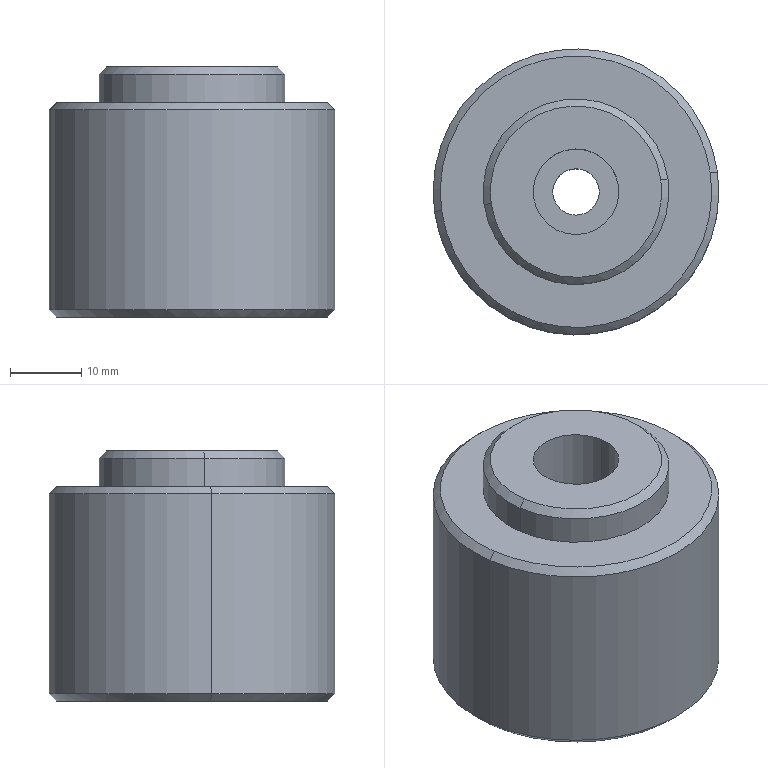Component | SolidWorks | TAR-02-030CoarseKnurledHandwheel-1 | 1 solid | 21 faces | box 40 x 40 x 35 mm | volume 37397 mm3 | cylinder 10 | cone 6 | plane 5 | commonest cylinder face diameters 11 x2 12 x2 26 x2 40 x2 6.5 x2
build123d program:
from build123d import *

# Parameters (mm, degrees)
SKETCH1_R           = 20
BOSS_EXTRUDE1_DEPTH = 30
SKETCH2_R           = 13
BOSS_EXTRUDE2_DEPTH = 5
SKETCH3_R           = 6
CUT_EXTRUDE1_DEPTH  = 15
SKETCH4_R           = 3.25
CUT_EXTRUDE2_DEPTH  = 99
SKETCH5_R           = 5.5
CUT_EXTRUDE3_DEPTH  = 7
CHAMFER1_SIZE       = 1


with BuildPart() as part:
    # Sketch1 → Boss-Extrude1 (new body)
    with BuildSketch(Plane.XY):
        Circle(SKETCH1_R)
    extrude(amount=BOSS_EXTRUDE1_DEPTH)

    # Sketch2 → Boss-Extrude2 (add)
    with BuildSketch(Plane.XY.offset(30)):
        Circle(SKETCH2_R)
    extrude(amount=BOSS_EXTRUDE2_DEPTH)

    # Sketch3 → Cut-Extrude1 (cut)
    with BuildSketch(Plane.XY.offset(35)):
        Circle(SKETCH3_R)
    extrude(amount=-CUT_EXTRUDE1_DEPTH, mode=Mode.SUBTRACT)

    # Sketch4 → Cut-Extrude2 (cut)
    with BuildSketch(Plane.XY.offset(20)):
        Circle(SKETCH4_R)
    extrude(amount=-CUT_EXTRUDE2_DEPTH, mode=Mode.SUBTRACT)

    # Sketch5 → Cut-Extrude3 (cut)
    with BuildSketch(Plane(origin=(0, 0, 0), x_dir=(-1, 0, 0), z_dir=(0, 0, -1))):
        Circle(SKETCH5_R)
    extrude(amount=-CUT_EXTRUDE3_DEPTH, mode=Mode.SUBTRACT)

    # Chamfer1
    chamfer1_edges = [part.edges().sort_by_distance(p)[0] for p in [
        (-20, 0, 0),
        (-20, 0, 30),
        (-13, 0, 35),
    ]]
    chamfer(chamfer1_edges, length=CHAMFER1_SIZE)


solid = part.part

# Placed as in the assembly
solid = solid.moved(Location((14.609, 9.288, -212.6), (0, 0, 0)))
STEP:
#1=COLOUR_RGB('',0.7922,0.8196,0.9333);
#2=FILL_AREA_STYLE_COLOUR('',#1);
#3=FILL_AREA_STYLE('',(#2));
#4=SURFACE_STYLE_FILL_AREA(#3);
#5=SURFACE_SIDE_STYLE('',(#4));
#6=SURFACE_STYLE_USAGE(.BOTH.,#5);
#7=PRESENTATION_STYLE_ASSIGNMENT((#6));
#8=CARTESIAN_POINT('',(1.043,0.4308,-6.992));
#9=VERTEX_POINT('',#8);
#10=CARTESIAN_POINT('',(0.1072,0.3005,-6.992));
#11=VERTEX_POINT('',#10);
#12=CARTESIAN_POINT('',(0.5752,0.3657,-6.992));
#13=DIRECTION('',(0.,0.,1.));
#14=DIRECTION('',(0.9904,0.1379,0.));
#15=AXIS2_PLACEMENT_3D('',#12,#13,#14);
#16=CIRCLE('',#15,0.4724);
#17=EDGE_CURVE('',#9,#11,#16,.T.);
#18=ORIENTED_EDGE('',*,*,#17,.F.);
#19=CARTESIAN_POINT('',(1.082,0.4362,-7.031));
#20=VERTEX_POINT('',#19);
#21=CARTESIAN_POINT('',(1.043,0.4308,-6.992));
#22=DIRECTION('',(0.7004,0.09749,-0.7071));
#23=VECTOR('',#22,39.37);
#24=LINE('',#21,#23);
#25=EDGE_CURVE('',#9,#20,#24,.T.);
#26=ORIENTED_EDGE('',*,*,#25,.T.);
#27=CARTESIAN_POINT('',(0.06824,0.2951,-7.031));
#28=VERTEX_POINT('',#27);
#29=CARTESIAN_POINT('',(0.5752,0.3657,-7.031));
#30=DIRECTION('',(0.,0.,-1.));
#31=DIRECTION('',(0.9904,0.1379,0.));
#32=AXIS2_PLACEMENT_3D('',#29,#30,#31);
#33=CIRCLE('',#32,0.5118);
#34=EDGE_CURVE('',#28,#20,#33,.T.);
#35=ORIENTED_EDGE('',*,*,#34,.F.);
#36=CARTESIAN_POINT('',(0.1072,0.3005,-6.992));
#37=DIRECTION('',(-0.7004,-0.09749,-0.7071));
#38=VECTOR('',#37,39.37);
#39=LINE('',#36,#38);
#40=EDGE_CURVE('',#11,#28,#39,.T.);
#41=ORIENTED_EDGE('',*,*,#40,.F.);
#42=EDGE_LOOP('',(#18,#26,#35,#41));
#43=FACE_OUTER_BOUND('',#42,.T.);
#44=CARTESIAN_POINT('',(0.5752,0.3657,-6.992));
#45=DIRECTION('',(0.,0.,-1.));
#46=DIRECTION('',(-0.9904,-0.1379,0.));
#47=AXIS2_PLACEMENT_3D('',#44,#45,#46);
#48=CONICAL_SURFACE('',#47,0.4724,0.7854);
#49=ADVANCED_FACE('',(#43),#48,.T.);
#50=CARTESIAN_POINT('',(1.316,0.4688,-7.189));
#51=VERTEX_POINT('',#50);
#52=CARTESIAN_POINT('',(-0.1657,0.2625,-7.189));
#53=VERTEX_POINT('',#52);
#54=CARTESIAN_POINT('',(0.5752,0.3657,-7.189));
#55=DIRECTION('',(0.,0.,1.));
#56=DIRECTION('',(0.9904,0.1379,0.));
#57=AXIS2_PLACEMENT_3D('',#54,#55,#56);
#58=CIRCLE('',#57,0.748);
#59=EDGE_CURVE('',#51,#53,#58,.T.);
#60=ORIENTED_EDGE('',*,*,#59,.F.);
#61=CARTESIAN_POINT('',(1.355,0.4742,-7.228));
#62=VERTEX_POINT('',#61);
#63=CARTESIAN_POINT('',(1.316,0.4688,-7.189));
#64=DIRECTION('',(0.7004,0.09749,-0.7071));
#65=VECTOR('',#64,39.37);
#66=LINE('',#63,#65);
#67=EDGE_CURVE('',#51,#62,#66,.T.);
#68=ORIENTED_EDGE('',*,*,#67,.T.);
#69=CARTESIAN_POINT('',(-0.2047,0.2571,-7.228));
#70=VERTEX_POINT('',#69);
#71=CARTESIAN_POINT('',(0.5752,0.3657,-7.228));
#72=DIRECTION('',(0.,0.,-1.));
#73=DIRECTION('',(0.9904,0.1379,0.));
#74=AXIS2_PLACEMENT_3D('',#71,#72,#73);
#75=CIRCLE('',#74,0.7874);
#76=EDGE_CURVE('',#70,#62,#75,.T.);
#77=ORIENTED_EDGE('',*,*,#76,.F.);
#78=CARTESIAN_POINT('',(-0.1657,0.2625,-7.189));
#79=DIRECTION('',(-0.7004,-0.09749,-0.7071));
#80=VECTOR('',#79,39.37);
#81=LINE('',#78,#80);
#82=EDGE_CURVE('',#53,#70,#81,.T.);
#83=ORIENTED_EDGE('',*,*,#82,.F.);
#84=EDGE_LOOP('',(#60,#68,#77,#83));
#85=FACE_OUTER_BOUND('',#84,.T.);
#86=CARTESIAN_POINT('',(0.5752,0.3657,-7.189));
#87=DIRECTION('',(0.,0.,-1.));
#88=DIRECTION('',(-0.9904,-0.1379,0.));
#89=AXIS2_PLACEMENT_3D('',#86,#87,#88);
#90=CONICAL_SURFACE('',#89,0.748,0.7854);
#91=ADVANCED_FACE('',(#85),#90,.T.);
#92=CARTESIAN_POINT('',(-0.1657,0.2625,-8.37));
#93=VERTEX_POINT('',#92);
#94=CARTESIAN_POINT('',(1.316,0.4688,-8.37));
#95=VERTEX_POINT('',#94);
#96=CARTESIAN_POINT('',(0.5752,0.3657,-8.37));
#97=DIRECTION('',(0.,0.,-1.));
#98=DIRECTION('',(0.9904,0.1379,0.));
#99=AXIS2_PLACEMENT_3D('',#96,#97,#98);
#100=CIRCLE('',#99,0.748);
#101=EDGE_CURVE('',#93,#95,#100,.T.);
#102=ORIENTED_EDGE('',*,*,#101,.F.);
#103=CARTESIAN_POINT('',(-0.2047,0.2571,-8.331));
#104=VERTEX_POINT('',#103);
#105=CARTESIAN_POINT('',(-0.2047,0.2571,-8.331));
#106=DIRECTION('',(-0.7004,-0.09749,0.7071));
#107=VECTOR('',#106,39.37);
#108=LINE('',#105,#107);
#109=EDGE_CURVE('',#93,#104,#108,.T.);
#110=ORIENTED_EDGE('',*,*,#109,.T.);
#111=CARTESIAN_POINT('',(1.355,0.4742,-8.331));
#112=VERTEX_POINT('',#111);
#113=CARTESIAN_POINT('',(0.5752,0.3657,-8.331));
#114=DIRECTION('',(0.,0.,1.));
#115=DIRECTION('',(0.9904,0.1379,0.));
#116=AXIS2_PLACEMENT_3D('',#113,#114,#115);
#117=CIRCLE('',#116,0.7874);
#118=EDGE_CURVE('',#112,#104,#117,.T.);
#119=ORIENTED_EDGE('',*,*,#118,.F.);
#120=CARTESIAN_POINT('',(1.355,0.4742,-8.331));
#121=DIRECTION('',(0.7004,0.09749,0.7071));
#122=VECTOR('',#121,39.37);
#123=LINE('',#120,#122);
#124=EDGE_CURVE('',#95,#112,#123,.T.);
#125=ORIENTED_EDGE('',*,*,#124,.F.);
#126=EDGE_LOOP('',(#102,#110,#119,#125));
#127=FACE_OUTER_BOUND('',#126,.T.);
#128=CARTESIAN_POINT('',(0.5752,0.3657,-8.331));
#129=DIRECTION('',(0.,0.,1.));
#130=DIRECTION('',(0.9904,0.1379,0.));
#131=AXIS2_PLACEMENT_3D('',#128,#129,#130);
#132=CONICAL_SURFACE('',#131,0.7874,0.7854);
#133=ADVANCED_FACE('',(#127),#132,.T.);
#134=CARTESIAN_POINT('',(0.7896,0.3955,-8.094));
#135=VERTEX_POINT('',#134);
#136=CARTESIAN_POINT('',(0.3607,0.3358,-8.094));
#137=VERTEX_POINT('',#136);
#138=CARTESIAN_POINT('',(0.5752,0.3657,-8.094));
#139=DIRECTION('',(0.,0.,-1.));
#140=DIRECTION('',(-0.9904,-0.1379,0.));
#141=AXIS2_PLACEMENT_3D('',#138,#139,#140);
#142=CIRCLE('',#141,0.2165);
#143=EDGE_CURVE('',#135,#137,#142,.T.);
#144=ORIENTED_EDGE('',*,*,#143,.F.);
#145=CARTESIAN_POINT('',(0.7896,0.3955,-8.37));
#146=VERTEX_POINT('',#145);
#147=CARTESIAN_POINT('',(0.7896,0.3955,-8.094));
#148=DIRECTION('',(0.,0.,-1.));
#149=VECTOR('',#148,39.37);
#150=LINE('',#147,#149);
#151=EDGE_CURVE('',#135,#146,#150,.T.);
#152=ORIENTED_EDGE('',*,*,#151,.T.);
#153=CARTESIAN_POINT('',(0.3607,0.3358,-8.37));
#154=VERTEX_POINT('',#153);
#155=CARTESIAN_POINT('',(0.5752,0.3657,-8.37));
#156=DIRECTION('',(0.,0.,-1.));
#157=DIRECTION('',(-0.9904,-0.1379,0.));
#158=AXIS2_PLACEMENT_3D('',#155,#156,#157);
#159=CIRCLE('',#158,0.2165);
#160=EDGE_CURVE('',#146,#154,#159,.T.);
#161=ORIENTED_EDGE('',*,*,#160,.T.);
#162=CARTESIAN_POINT('',(0.3607,0.3358,-8.094));
#163=DIRECTION('',(0.,0.,-1.));
#164=VECTOR('',#163,39.37);
#165=LINE('',#162,#164);
#166=EDGE_CURVE('',#137,#154,#165,.T.);
#167=ORIENTED_EDGE('',*,*,#166,.F.);
#168=EDGE_LOOP('',(#144,#152,#161,#167));
#169=FACE_OUTER_BOUND('',#168,.T.);
#170=CARTESIAN_POINT('',(0.5752,0.3657,-8.094));
#171=DIRECTION('',(0.,0.,-1.));
#172=DIRECTION('',(-0.9904,-0.1379,0.));
#173=AXIS2_PLACEMENT_3D('',#170,#171,#172);
#174=CYLINDRICAL_SURFACE('',#173,0.2165);
#175=ADVANCED_FACE('',(#169),#174,.F.);
#176=CARTESIAN_POINT('',(0.3412,0.3331,-7.583));
#177=VERTEX_POINT('',#176);
#178=CARTESIAN_POINT('',(0.8091,0.3982,-7.583));
#179=VERTEX_POINT('',#178);
#180=CARTESIAN_POINT('',(0.5752,0.3657,-7.583));
#181=DIRECTION('',(0.,0.,1.));
#182=DIRECTION('',(0.9904,0.1379,0.));
#183=AXIS2_PLACEMENT_3D('',#180,#181,#182);
#184=CIRCLE('',#183,0.2362);
#185=EDGE_CURVE('',#177,#179,#184,.T.);
#186=ORIENTED_EDGE('',*,*,#185,.F.);
#187=CARTESIAN_POINT('',(0.3412,0.3331,-6.992));
#188=VERTEX_POINT('',#187);
#189=CARTESIAN_POINT('',(0.3412,0.3331,-7.583));
#190=DIRECTION('',(0.,0.,1.));
#191=VECTOR('',#190,39.37);
#192=LINE('',#189,#191);
#193=EDGE_CURVE('',#177,#188,#192,.T.);
#194=ORIENTED_EDGE('',*,*,#193,.T.);
#195=CARTESIAN_POINT('',(0.8091,0.3982,-6.992));
#196=VERTEX_POINT('',#195);
#197=CARTESIAN_POINT('',(0.5752,0.3657,-6.992));
#198=DIRECTION('',(0.,0.,1.));
#199=DIRECTION('',(0.9904,0.1379,0.));
#200=AXIS2_PLACEMENT_3D('',#197,#198,#199);
#201=CIRCLE('',#200,0.2362);
#202=EDGE_CURVE('',#188,#196,#201,.T.);
#203=ORIENTED_EDGE('',*,*,#202,.T.);
#204=CARTESIAN_POINT('',(0.8091,0.3982,-7.583));
#205=DIRECTION('',(0.,0.,1.));
#206=VECTOR('',#205,39.37);
#207=LINE('',#204,#206);
#208=EDGE_CURVE('',#179,#196,#207,.T.);
#209=ORIENTED_EDGE('',*,*,#208,.F.);
#210=EDGE_LOOP('',(#186,#194,#203,#209));
#211=FACE_OUTER_BOUND('',#210,.T.);
#212=CARTESIAN_POINT('',(0.5752,0.3657,-7.583));
#213=DIRECTION('',(0.,0.,1.));
#214=DIRECTION('',(0.9904,0.1379,0.));
#215=AXIS2_PLACEMENT_3D('',#212,#213,#214);
#216=CYLINDRICAL_SURFACE('',#215,0.2362);
#217=ADVANCED_FACE('',(#211),#216,.F.);
#218=ORIENTED_EDGE('',*,*,#34,.T.);
#219=CARTESIAN_POINT('',(1.082,0.4362,-7.189));
#220=VERTEX_POINT('',#219);
#221=CARTESIAN_POINT('',(1.082,0.4362,-6.992));
#222=DIRECTION('',(0.,0.,-1.));
#223=VECTOR('',#222,39.37);
#224=LINE('',#221,#223);
#225=EDGE_CURVE('',#20,#220,#224,.T.);
#226=ORIENTED_EDGE('',*,*,#225,.T.);
#227=CARTESIAN_POINT('',(0.06824,0.2951,-7.189));
#228=VERTEX_POINT('',#227);
#229=CARTESIAN_POINT('',(0.5752,0.3657,-7.189));
#230=DIRECTION('',(0.,0.,1.));
#231=DIRECTION('',(0.9904,0.1379,0.));
#232=AXIS2_PLACEMENT_3D('',#229,#230,#231);
#233=CIRCLE('',#232,0.5118);
#234=EDGE_CURVE('',#220,#228,#233,.T.);
#235=ORIENTED_EDGE('',*,*,#234,.T.);
#236=CARTESIAN_POINT('',(0.06824,0.2951,-6.992));
#237=DIRECTION('',(0.,0.,-1.));
#238=VECTOR('',#237,39.37);
#239=LINE('',#236,#238);
#240=EDGE_CURVE('',#28,#228,#239,.T.);
#241=ORIENTED_EDGE('',*,*,#240,.F.);
#242=EDGE_LOOP('',(#218,#226,#235,#241));
#243=FACE_OUTER_BOUND('',#242,.T.);
#244=CARTESIAN_POINT('',(0.5752,0.3657,-6.992));
#245=DIRECTION('',(0.,0.,-1.));
#246=DIRECTION('',(-0.9904,-0.1379,0.));
#247=AXIS2_PLACEMENT_3D('',#244,#245,#246);
#248=CYLINDRICAL_SURFACE('',#247,0.5118);
#249=ADVANCED_FACE('',(#243),#248,.T.);
#250=ORIENTED_EDGE('',*,*,#76,.T.);
#251=CARTESIAN_POINT('',(1.355,0.4742,-7.189));
#252=DIRECTION('',(0.,0.,-1.));
#253=VECTOR('',#252,39.37);
#254=LINE('',#251,#253);
#255=EDGE_CURVE('',#62,#112,#254,.T.);
#256=ORIENTED_EDGE('',*,*,#255,.T.);
#257=ORIENTED_EDGE('',*,*,#118,.T.);
#258=CARTESIAN_POINT('',(-0.2047,0.2571,-7.189));
#259=DIRECTION('',(0.,0.,-1.));
#260=VECTOR('',#259,39.37);
#261=LINE('',#258,#260);
#262=EDGE_CURVE('',#70,#104,#261,.T.);
#263=ORIENTED_EDGE('',*,*,#262,.F.);
#264=EDGE_LOOP('',(#250,#256,#257,#263));
#265=FACE_OUTER_BOUND('',#264,.T.);
#266=CARTESIAN_POINT('',(0.5752,0.3657,-7.189));
#267=DIRECTION('',(0.,0.,-1.));
#268=DIRECTION('',(-0.9904,-0.1379,0.));
#269=AXIS2_PLACEMENT_3D('',#266,#267,#268);
#270=CYLINDRICAL_SURFACE('',#269,0.7874);
#271=ADVANCED_FACE('',(#265),#270,.T.);
#272=CARTESIAN_POINT('',(0.4484,0.348,-8.094));
#273=VERTEX_POINT('',#272);
#274=CARTESIAN_POINT('',(0.7019,0.3833,-8.094));
#275=VERTEX_POINT('',#274);
#276=CARTESIAN_POINT('',(0.5752,0.3657,-8.094));
#277=DIRECTION('',(0.,0.,1.));
#278=DIRECTION('',(-0.9904,-0.1379,0.));
#279=AXIS2_PLACEMENT_3D('',#276,#277,#278);
#280=CIRCLE('',#279,0.128);
#281=EDGE_CURVE('',#273,#275,#280,.T.);
#282=ORIENTED_EDGE('',*,*,#281,.F.);
#283=CARTESIAN_POINT('',(0.4484,0.348,-7.583));
#284=VERTEX_POINT('',#283);
#285=CARTESIAN_POINT('',(0.4484,0.348,-11.48));
#286=DIRECTION('',(0.,0.,1.));
#287=VECTOR('',#286,39.37);
#288=LINE('',#285,#287);
#289=EDGE_CURVE('',#273,#284,#288,.T.);
#290=ORIENTED_EDGE('',*,*,#289,.T.);
#291=CARTESIAN_POINT('',(0.7019,0.3833,-7.583));
#292=VERTEX_POINT('',#291);
#293=CARTESIAN_POINT('',(0.5752,0.3657,-7.583));
#294=DIRECTION('',(0.,0.,1.));
#295=DIRECTION('',(0.9904,0.1379,0.));
#296=AXIS2_PLACEMENT_3D('',#293,#294,#295);
#297=CIRCLE('',#296,0.128);
#298=EDGE_CURVE('',#284,#292,#297,.T.);
#299=ORIENTED_EDGE('',*,*,#298,.T.);
#300=CARTESIAN_POINT('',(0.7019,0.3833,-11.48));
#301=DIRECTION('',(0.,0.,1.));
#302=VECTOR('',#301,39.37);
#303=LINE('',#300,#302);
#304=EDGE_CURVE('',#275,#292,#303,.T.);
#305=ORIENTED_EDGE('',*,*,#304,.F.);
#306=EDGE_LOOP('',(#282,#290,#299,#305));
#307=FACE_OUTER_BOUND('',#306,.T.);
#308=CARTESIAN_POINT('',(0.5752,0.3657,-11.48));
#309=DIRECTION('',(0.,0.,1.));
#310=DIRECTION('',(0.9904,0.1379,0.));
#311=AXIS2_PLACEMENT_3D('',#308,#309,#310);
#312=CYLINDRICAL_SURFACE('',#311,0.128);
#313=ADVANCED_FACE('',(#307),#312,.F.);
#314=ORIENTED_EDGE('',*,*,#289,.F.);
#315=CARTESIAN_POINT('',(0.5752,0.3657,-8.094));
#316=DIRECTION('',(0.,0.,1.));
#317=DIRECTION('',(-0.9904,-0.1379,0.));
#318=AXIS2_PLACEMENT_3D('',#315,#316,#317);
#319=CIRCLE('',#318,0.128);
#320=EDGE_CURVE('',#275,#273,#319,.T.);
#321=ORIENTED_EDGE('',*,*,#320,.F.);
#322=ORIENTED_EDGE('',*,*,#304,.T.);
#323=CARTESIAN_POINT('',(0.5752,0.3657,-7.583));
#324=DIRECTION('',(0.,0.,1.));
#325=DIRECTION('',(0.9904,0.1379,0.));
#326=AXIS2_PLACEMENT_3D('',#323,#324,#325);
#327=CIRCLE('',#326,0.128);
#328=EDGE_CURVE('',#292,#284,#327,.T.);
#329=ORIENTED_EDGE('',*,*,#328,.T.);
#330=EDGE_LOOP('',(#314,#321,#322,#329));
#331=FACE_OUTER_BOUND('',#330,.T.);
#332=CARTESIAN_POINT('',(0.5752,0.3657,-11.48));
#333=DIRECTION('',(0.,0.,1.));
#334=DIRECTION('',(0.9904,0.1379,0.));
#335=AXIS2_PLACEMENT_3D('',#332,#333,#334);
#336=CYLINDRICAL_SURFACE('',#335,0.128);
#337=ADVANCED_FACE('',(#331),#336,.F.);
#338=ORIENTED_EDGE('',*,*,#255,.F.);
#339=CARTESIAN_POINT('',(0.5752,0.3657,-7.228));
#340=DIRECTION('',(0.,0.,-1.));
#341=DIRECTION('',(0.9904,0.1379,0.));
#342=AXIS2_PLACEMENT_3D('',#339,#340,#341);
#343=CIRCLE('',#342,0.7874);
#344=EDGE_CURVE('',#62,#70,#343,.T.);
#345=ORIENTED_EDGE('',*,*,#344,.T.);
#346=ORIENTED_EDGE('',*,*,#262,.T.);
#347=CARTESIAN_POINT('',(0.5752,0.3657,-8.331));
#348=DIRECTION('',(0.,0.,1.));
#349=DIRECTION('',(0.9904,0.1379,0.));
#350=AXIS2_PLACEMENT_3D('',#347,#348,#349);
#351=CIRCLE('',#350,0.7874);
#352=EDGE_CURVE('',#104,#112,#351,.T.);
#353=ORIENTED_EDGE('',*,*,#352,.T.);
#354=EDGE_LOOP('',(#338,#345,#346,#353));
#355=FACE_OUTER_BOUND('',#354,.T.);
#356=CARTESIAN_POINT('',(0.5752,0.3657,-7.189));
#357=DIRECTION('',(0.,0.,-1.));
#358=DIRECTION('',(-0.9904,-0.1379,0.));
#359=AXIS2_PLACEMENT_3D('',#356,#357,#358);
#360=CYLINDRICAL_SURFACE('',#359,0.7874);
#361=ADVANCED_FACE('',(#355),#360,.T.);
#362=CARTESIAN_POINT('',(0.5752,0.3657,-7.189));
#363=DIRECTION('',(0.,0.,1.));
#364=DIRECTION('',(0.9904,0.1379,0.));
#365=AXIS2_PLACEMENT_3D('',#362,#363,#364);
#366=CIRCLE('',#365,0.748);
#367=EDGE_CURVE('',#53,#51,#366,.T.);
#368=ORIENTED_EDGE('',*,*,#367,.T.);
#369=ORIENTED_EDGE('',*,*,#59,.T.);
#370=EDGE_LOOP('',(#368,#369));
#371=FACE_OUTER_BOUND('',#370,.T.);
#372=CARTESIAN_POINT('',(0.5752,0.3657,-7.189));
#373=DIRECTION('',(0.,0.,1.));
#374=DIRECTION('',(0.9904,0.1379,0.));
#375=AXIS2_PLACEMENT_3D('',#372,#373,#374);
#376=CIRCLE('',#375,0.5118);
#377=EDGE_CURVE('',#228,#220,#376,.T.);
#378=ORIENTED_EDGE('',*,*,#377,.F.);
#379=ORIENTED_EDGE('',*,*,#234,.F.);
#380=EDGE_LOOP('',(#378,#379));
#381=FACE_BOUND('',#380,.T.);
#382=CARTESIAN_POINT('',(0.5752,0.3657,-7.189));
#383=DIRECTION('',(0.,0.,1.));
#384=DIRECTION('',(0.9904,0.1379,0.));
#385=AXIS2_PLACEMENT_3D('',#382,#383,#384);
#386=PLANE('',#385);
#387=ADVANCED_FACE('',(#371,#381),#386,.T.);
#388=CARTESIAN_POINT('',(0.5752,0.3657,-8.37));
#389=DIRECTION('',(0.,0.,-1.));
#390=DIRECTION('',(0.9904,0.1379,0.));
#391=AXIS2_PLACEMENT_3D('',#388,#389,#390);
#392=CIRCLE('',#391,0.748);
#393=EDGE_CURVE('',#95,#93,#392,.T.);
#394=ORIENTED_EDGE('',*,*,#393,.T.);
#395=ORIENTED_EDGE('',*,*,#101,.T.);
#396=EDGE_LOOP('',(#394,#395));
#397=FACE_OUTER_BOUND('',#396,.T.);
#398=CARTESIAN_POINT('',(0.5752,0.3657,-8.37));
#399=DIRECTION('',(0.,0.,-1.));
#400=DIRECTION('',(-0.9904,-0.1379,0.));
#401=AXIS2_PLACEMENT_3D('',#398,#399,#400);
#402=CIRCLE('',#401,0.2165);
#403=EDGE_CURVE('',#154,#146,#402,.T.);
#404=ORIENTED_EDGE('',*,*,#403,.F.);
#405=ORIENTED_EDGE('',*,*,#160,.F.);
#406=EDGE_LOOP('',(#404,#405));
#407=FACE_BOUND('',#406,.T.);
#408=CARTESIAN_POINT('',(0.5752,0.3657,-8.37));
#409=DIRECTION('',(0.,0.,1.));
#410=DIRECTION('',(0.9904,0.1379,0.));
#411=AXIS2_PLACEMENT_3D('',#408,#409,#410);
#412=PLANE('',#411);
#413=ADVANCED_FACE('',(#397,#407),#412,.F.);
#414=ORIENTED_EDGE('',*,*,#225,.F.);
#415=CARTESIAN_POINT('',(0.5752,0.3657,-7.031));
#416=DIRECTION('',(0.,0.,-1.));
#417=DIRECTION('',(0.9904,0.1379,0.));
#418=AXIS2_PLACEMENT_3D('',#415,#416,#417);
#419=CIRCLE('',#418,0.5118);
#420=EDGE_CURVE('',#20,#28,#419,.T.);
#421=ORIENTED_EDGE('',*,*,#420,.T.);
#422=ORIENTED_EDGE('',*,*,#240,.T.);
#423=ORIENTED_EDGE('',*,*,#377,.T.);
#424=EDGE_LOOP('',(#414,#421,#422,#423));
#425=FACE_OUTER_BOUND('',#424,.T.);
#426=CARTESIAN_POINT('',(0.5752,0.3657,-6.992));
#427=DIRECTION('',(0.,0.,-1.));
#428=DIRECTION('',(-0.9904,-0.1379,0.));
#429=AXIS2_PLACEMENT_3D('',#426,#427,#428);
#430=CYLINDRICAL_SURFACE('',#429,0.5118);
#431=ADVANCED_FACE('',(#425),#430,.T.);
#432=CARTESIAN_POINT('',(0.5752,0.3657,-6.992));
#433=DIRECTION('',(0.,0.,1.));
#434=DIRECTION('',(0.9904,0.1379,0.));
#435=AXIS2_PLACEMENT_3D('',#432,#433,#434);
#436=CIRCLE('',#435,0.4724);
#437=EDGE_CURVE('',#11,#9,#436,.T.);
#438=ORIENTED_EDGE('',*,*,#437,.T.);
#439=ORIENTED_EDGE('',*,*,#17,.T.);
#440=EDGE_LOOP('',(#438,#439));
#441=FACE_OUTER_BOUND('',#440,.T.);
#442=CARTESIAN_POINT('',(0.5752,0.3657,-6.992));
#443=DIRECTION('',(0.,0.,1.));
#444=DIRECTION('',(0.9904,0.1379,0.));
#445=AXIS2_PLACEMENT_3D('',#442,#443,#444);
#446=CIRCLE('',#445,0.2362);
#447=EDGE_CURVE('',#196,#188,#446,.T.);
#448=ORIENTED_EDGE('',*,*,#447,.F.);
#449=ORIENTED_EDGE('',*,*,#202,.F.);
#450=EDGE_LOOP('',(#448,#449));
#451=FACE_BOUND('',#450,.T.);
#452=CARTESIAN_POINT('',(0.5752,0.3657,-6.992));
#453=DIRECTION('',(0.,0.,1.));
#454=DIRECTION('',(0.9904,0.1379,0.));
#455=AXIS2_PLACEMENT_3D('',#452,#453,#454);
#456=PLANE('',#455);
#457=ADVANCED_FACE('',(#441,#451),#456,.T.);
#458=ORIENTED_EDGE('',*,*,#193,.F.);
#459=CARTESIAN_POINT('',(0.5752,0.3657,-7.583));
#460=DIRECTION('',(0.,0.,1.));
#461=DIRECTION('',(0.9904,0.1379,0.));
#462=AXIS2_PLACEMENT_3D('',#459,#460,#461);
#463=CIRCLE('',#462,0.2362);
#464=EDGE_CURVE('',#179,#177,#463,.T.);
#465=ORIENTED_EDGE('',*,*,#464,.F.);
#466=ORIENTED_EDGE('',*,*,#208,.T.);
#467=ORIENTED_EDGE('',*,*,#447,.T.);
#468=EDGE_LOOP('',(#458,#465,#466,#467));
#469=FACE_OUTER_BOUND('',#468,.T.);
#470=CARTESIAN_POINT('',(0.5752,0.3657,-7.583));
#471=DIRECTION('',(0.,0.,1.));
#472=DIRECTION('',(0.9904,0.1379,0.));
#473=AXIS2_PLACEMENT_3D('',#470,#471,#472);
#474=CYLINDRICAL_SURFACE('',#473,0.2362);
#475=ADVANCED_FACE('',(#469),#474,.F.);
#476=ORIENTED_EDGE('',*,*,#328,.F.);
#477=ORIENTED_EDGE('',*,*,#298,.F.);
#478=EDGE_LOOP('',(#476,#477));
#479=FACE_BOUND('',#478,.T.);
#480=ORIENTED_EDGE('',*,*,#464,.T.);
#481=ORIENTED_EDGE('',*,*,#185,.T.);
#482=EDGE_LOOP('',(#480,#481));
#483=FACE_OUTER_BOUND('',#482,.T.);
#484=CARTESIAN_POINT('',(0.5752,0.3657,-7.583));
#485=DIRECTION('',(0.,0.,1.));
#486=DIRECTION('',(0.9904,0.1379,0.));
#487=AXIS2_PLACEMENT_3D('',#484,#485,#486);
#488=PLANE('',#487);
#489=ADVANCED_FACE('',(#479,#483),#488,.T.);
#490=CARTESIAN_POINT('',(0.5752,0.3657,-8.094));
#491=DIRECTION('',(0.,0.,-1.));
#492=DIRECTION('',(-0.9904,-0.1379,0.));
#493=AXIS2_PLACEMENT_3D('',#490,#491,#492);
#494=CIRCLE('',#493,0.2165);
#495=EDGE_CURVE('',#137,#135,#494,.T.);
#496=ORIENTED_EDGE('',*,*,#495,.T.);
#497=ORIENTED_EDGE('',*,*,#143,.T.);
#498=EDGE_LOOP('',(#496,#497));
#499=FACE_OUTER_BOUND('',#498,.T.);
#500=ORIENTED_EDGE('',*,*,#320,.T.);
#501=ORIENTED_EDGE('',*,*,#281,.T.);
#502=EDGE_LOOP('',(#500,#501));
#503=FACE_BOUND('',#502,.T.);
#504=CARTESIAN_POINT('',(0.5752,0.3657,-8.094));
#505=DIRECTION('',(0.,0.,-1.));
#506=DIRECTION('',(-0.9904,-0.1379,0.));
#507=AXIS2_PLACEMENT_3D('',#504,#505,#506);
#508=PLANE('',#507);
#509=ADVANCED_FACE('',(#499,#503),#508,.T.);
#510=ORIENTED_EDGE('',*,*,#151,.F.);
#511=ORIENTED_EDGE('',*,*,#495,.F.);
#512=ORIENTED_EDGE('',*,*,#166,.T.);
#513=ORIENTED_EDGE('',*,*,#403,.T.);
#514=EDGE_LOOP('',(#510,#511,#512,#513));
#515=FACE_OUTER_BOUND('',#514,.T.);
#516=CARTESIAN_POINT('',(0.5752,0.3657,-8.094));
#517=DIRECTION('',(0.,0.,-1.));
#518=DIRECTION('',(-0.9904,-0.1379,0.));
#519=AXIS2_PLACEMENT_3D('',#516,#517,#518);
#520=CYLINDRICAL_SURFACE('',#519,0.2165);
#521=ADVANCED_FACE('',(#515),#520,.F.);
#522=ORIENTED_EDGE('',*,*,#109,.F.);
#523=ORIENTED_EDGE('',*,*,#393,.F.);
#524=ORIENTED_EDGE('',*,*,#124,.T.);
#525=ORIENTED_EDGE('',*,*,#352,.F.);
#526=EDGE_LOOP('',(#522,#523,#524,#525));
#527=FACE_OUTER_BOUND('',#526,.T.);
#528=CARTESIAN_POINT('',(0.5752,0.3657,-8.331));
#529=DIRECTION('',(0.,0.,1.));
#530=DIRECTION('',(0.9904,0.1379,0.));
#531=AXIS2_PLACEMENT_3D('',#528,#529,#530);
#532=CONICAL_SURFACE('',#531,0.7874,0.7854);
#533=ADVANCED_FACE('',(#527),#532,.T.);
#534=ORIENTED_EDGE('',*,*,#67,.F.);
#535=ORIENTED_EDGE('',*,*,#367,.F.);
#536=ORIENTED_EDGE('',*,*,#82,.T.);
#537=ORIENTED_EDGE('',*,*,#344,.F.);
#538=EDGE_LOOP('',(#534,#535,#536,#537));
#539=FACE_OUTER_BOUND('',#538,.T.);
#540=CARTESIAN_POINT('',(0.5752,0.3657,-7.189));
#541=DIRECTION('',(0.,0.,-1.));
#542=DIRECTION('',(-0.9904,-0.1379,0.));
#543=AXIS2_PLACEMENT_3D('',#540,#541,#542);
#544=CONICAL_SURFACE('',#543,0.748,0.7854);
#545=ADVANCED_FACE('',(#539),#544,.T.);
#546=ORIENTED_EDGE('',*,*,#25,.F.);
#547=ORIENTED_EDGE('',*,*,#437,.F.);
#548=ORIENTED_EDGE('',*,*,#40,.T.);
#549=ORIENTED_EDGE('',*,*,#420,.F.);
#550=EDGE_LOOP('',(#546,#547,#548,#549));
#551=FACE_OUTER_BOUND('',#550,.T.);
#552=CARTESIAN_POINT('',(0.5752,0.3657,-6.992));
#553=DIRECTION('',(0.,0.,-1.));
#554=DIRECTION('',(-0.9904,-0.1379,0.));
#555=AXIS2_PLACEMENT_3D('',#552,#553,#554);
#556=CONICAL_SURFACE('',#555,0.4724,0.7854);
#557=ADVANCED_FACE('',(#551),#556,.T.);
#558=CLOSED_SHELL('',(#49,#91,#133,#175,#217,#249,#271,#313,#337,#361,#387,#413,#431,#457,#475,#489,#509,#521,#533,#545,#557));
#559=MANIFOLD_SOLID_BREP('',#558);
#560=STYLED_ITEM('',(#7),#559);
#561=PRESENTATION_LAYER_ASSIGNMENT('','',(#560));
#562=CARTESIAN_POINT('',(0.,0.,0.));
#563=DIRECTION('',(0.,0.,1.));
#564=DIRECTION('',(1.,0.,0.));
#565=AXIS2_PLACEMENT_3D('',#562,#563,#564);
#566=(LENGTH_UNIT()NAMED_UNIT(*)SI_UNIT($,.METRE.));
#567=LENGTH_MEASURE_WITH_UNIT(LENGTH_MEASURE(0.0254),#566);
#568=DIMENSIONAL_EXPONENTS(1.,0.,0.,0.,0.,0.,0.);
#569=(CONVERSION_BASED_UNIT('',#567)LENGTH_UNIT()NAMED_UNIT(#568));
#570=UNCERTAINTY_MEASURE_WITH_UNIT(LENGTH_MEASURE(0.00001),#569,'','');
#571=(NAMED_UNIT(*)PLANE_ANGLE_UNIT()SI_UNIT($,.RADIAN.));
#572=(NAMED_UNIT(*)SI_UNIT($,.STERADIAN.)SOLID_ANGLE_UNIT());
#573=(GEOMETRIC_REPRESENTATION_CONTEXT(3)GLOBAL_UNCERTAINTY_ASSIGNED_CONTEXT((#570))GLOBAL_UNIT_ASSIGNED_CONTEXT((#569,#571,#572))REPRESENTATION_CONTEXT('',''));
#574=ADVANCED_BREP_SHAPE_REPRESENTATION('',(#559,#565),#573);
#575=(LENGTH_UNIT()NAMED_UNIT(*)SI_UNIT($,.METRE.));
#576=LENGTH_MEASURE_WITH_UNIT(LENGTH_MEASURE(0.0254),#575);
#577=DIMENSIONAL_EXPONENTS(1.,0.,0.,0.,0.,0.,0.);
#578=(CONVERSION_BASED_UNIT('',#576)LENGTH_UNIT()NAMED_UNIT(#577));
#579=UNCERTAINTY_MEASURE_WITH_UNIT(LENGTH_MEASURE(0.00001),#578,'','');
#580=(NAMED_UNIT(*)PLANE_ANGLE_UNIT()SI_UNIT($,.RADIAN.));
#581=(NAMED_UNIT(*)SI_UNIT($,.STERADIAN.)SOLID_ANGLE_UNIT());
#582=(GEOMETRIC_REPRESENTATION_CONTEXT(3)GLOBAL_UNCERTAINTY_ASSIGNED_CONTEXT((#579))GLOBAL_UNIT_ASSIGNED_CONTEXT((#578,#580,#581))REPRESENTATION_CONTEXT('',''));
#583=MECHANICAL_DESIGN_GEOMETRIC_PRESENTATION_REPRESENTATION('',(#560),#582);